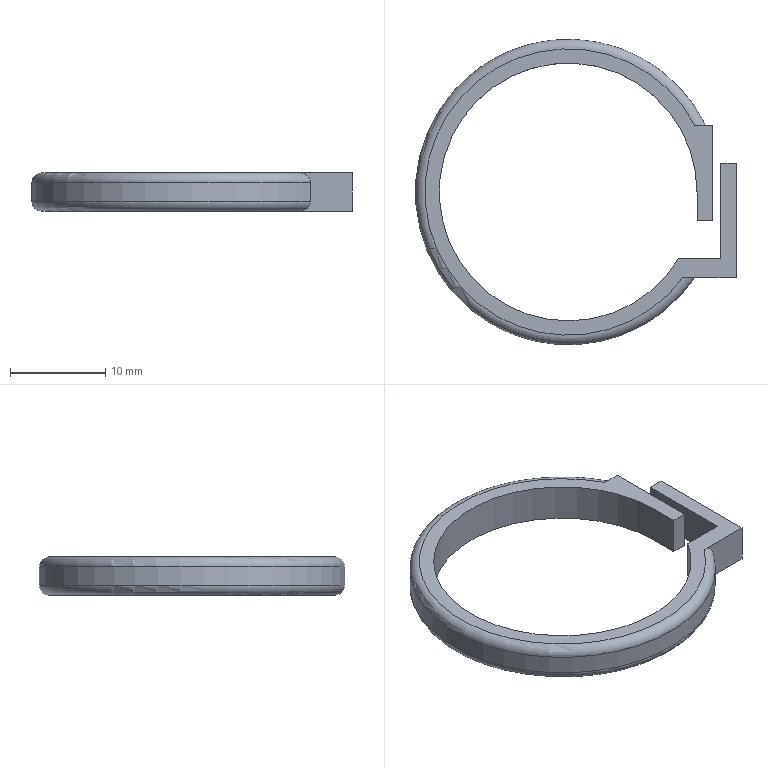Component | NX | CLAMP_2 | 1 solid | 15 faces | volume 921 mm3 | plane 11 | cylinder 2 | torus 2 | commonest cylinder face diameters 27 x1 32 x1